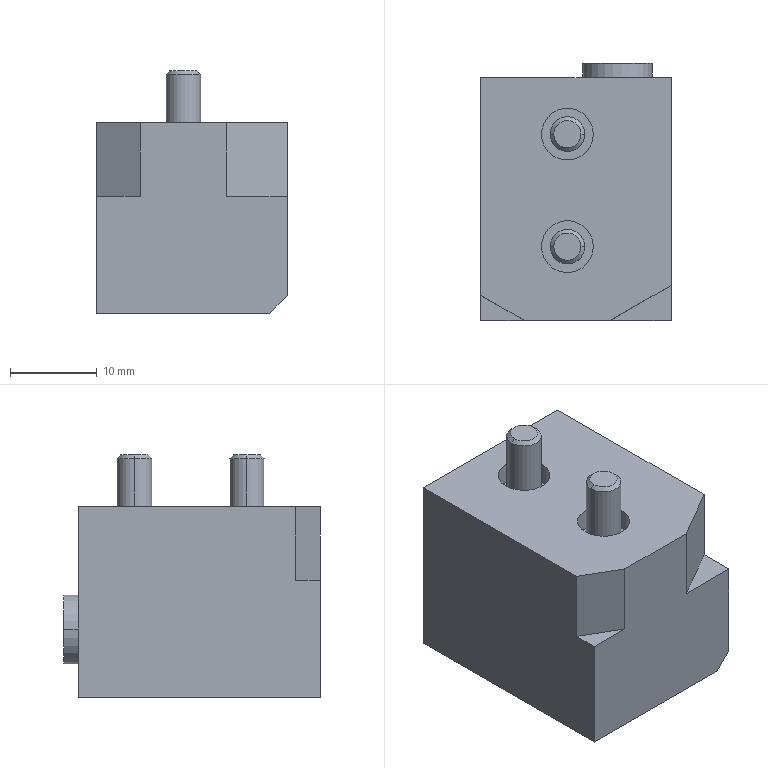Component | SolidWorks | SCHUNK-0303023 BSWS-B 64-1 | 1 solid | 43 faces | volume 11538 mm3 | plane 25 | cylinder 14 | cone 4 | commonest cylinder face diameters 6 x4 9 x4 4 x4 8 x2 | material Q235-A